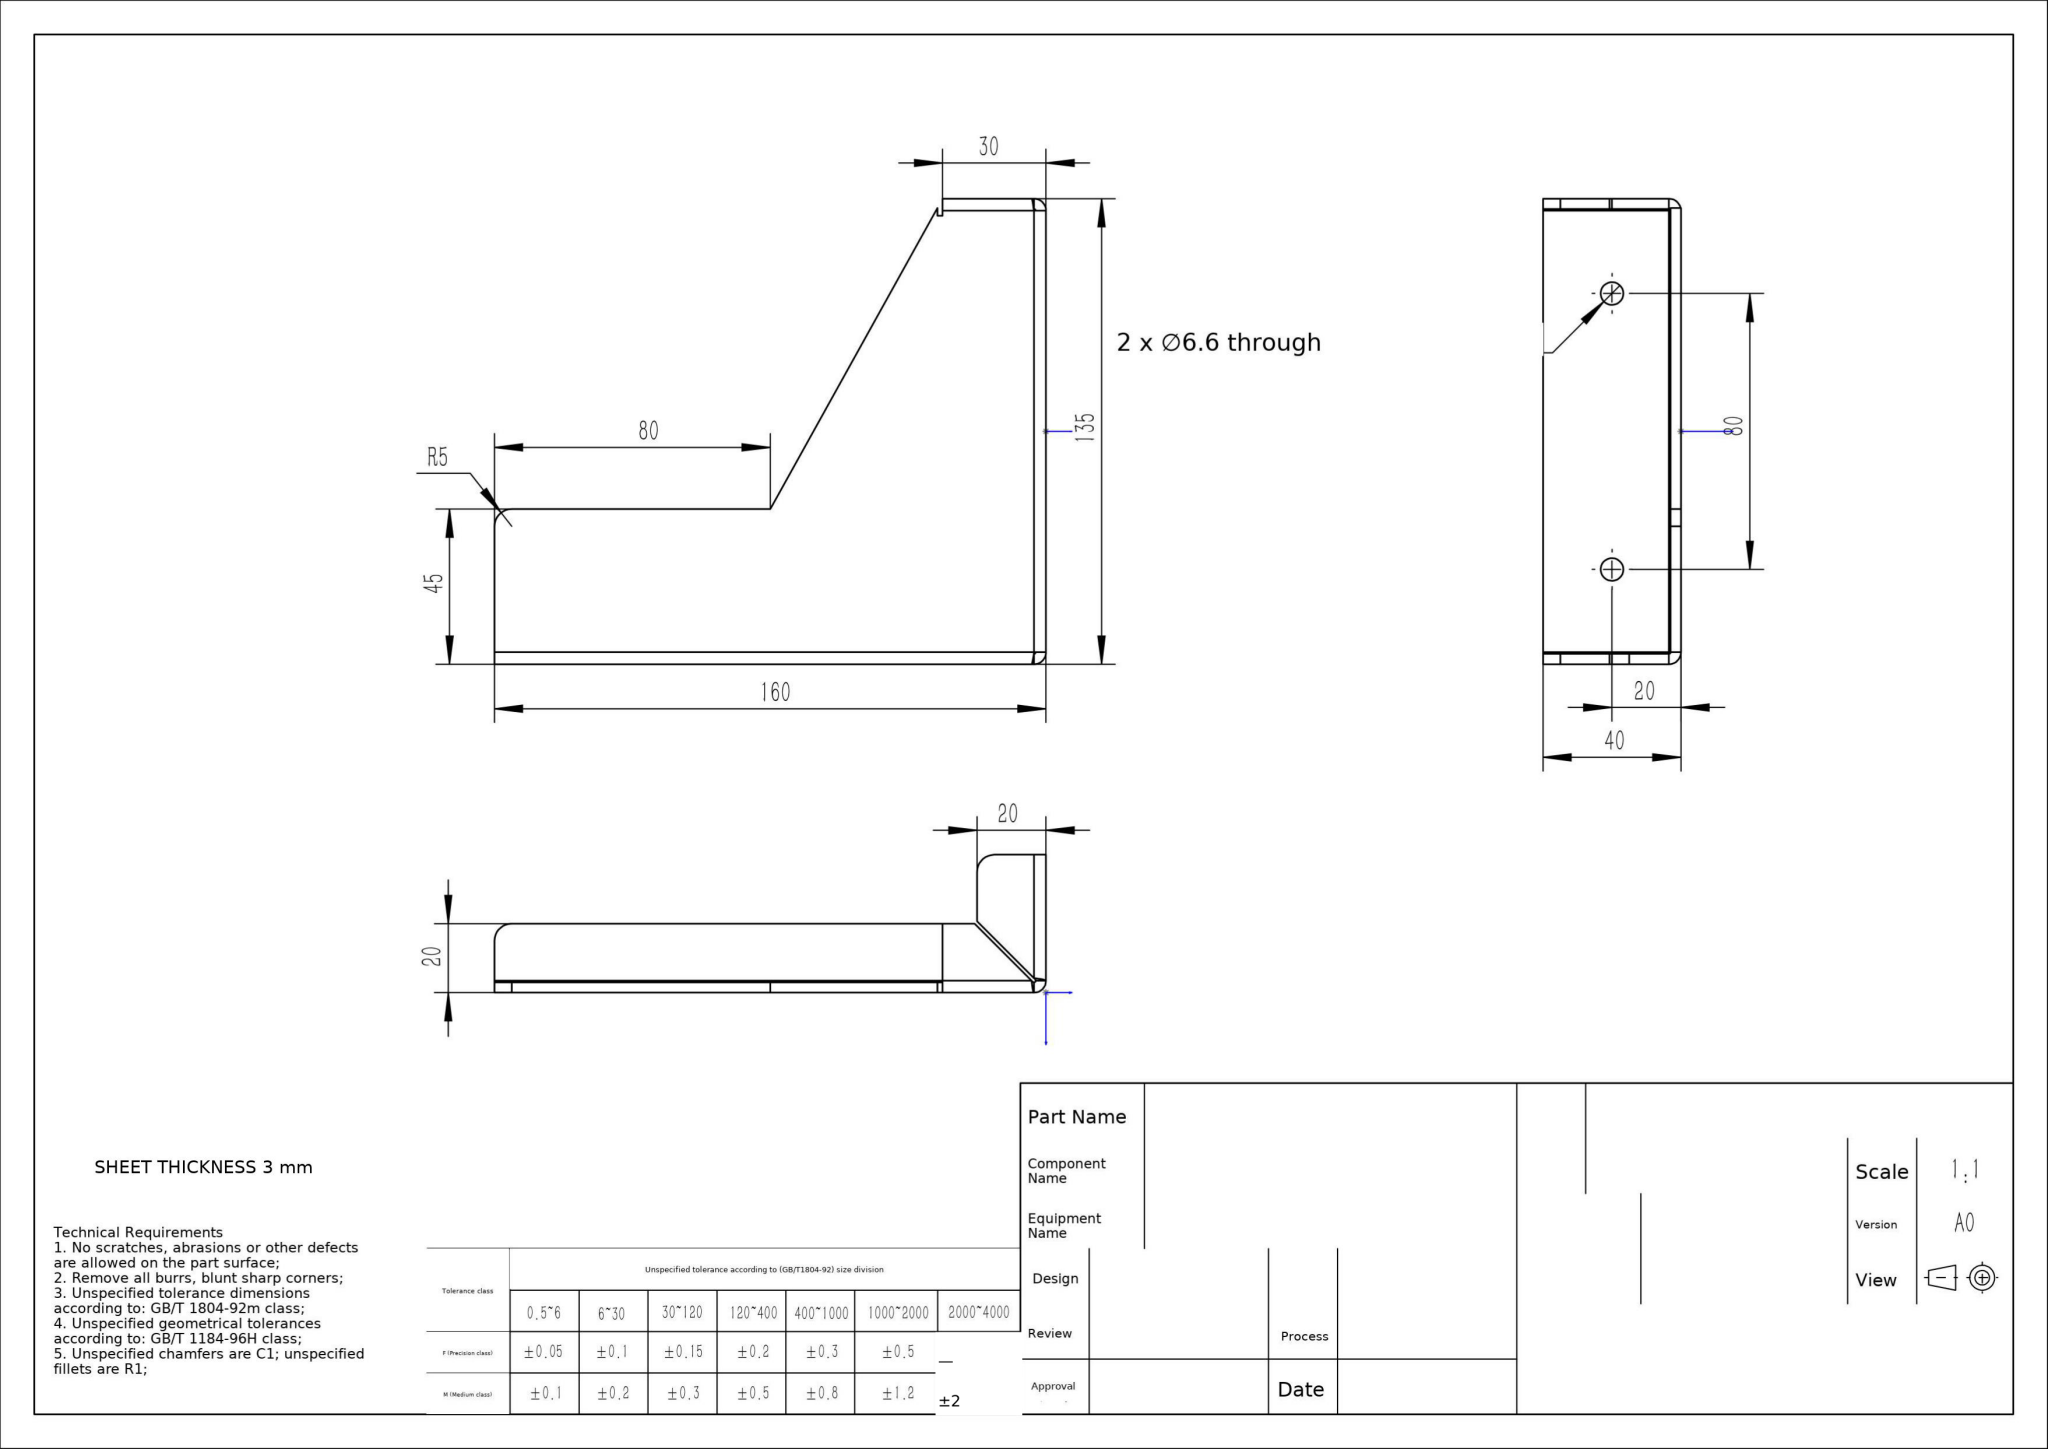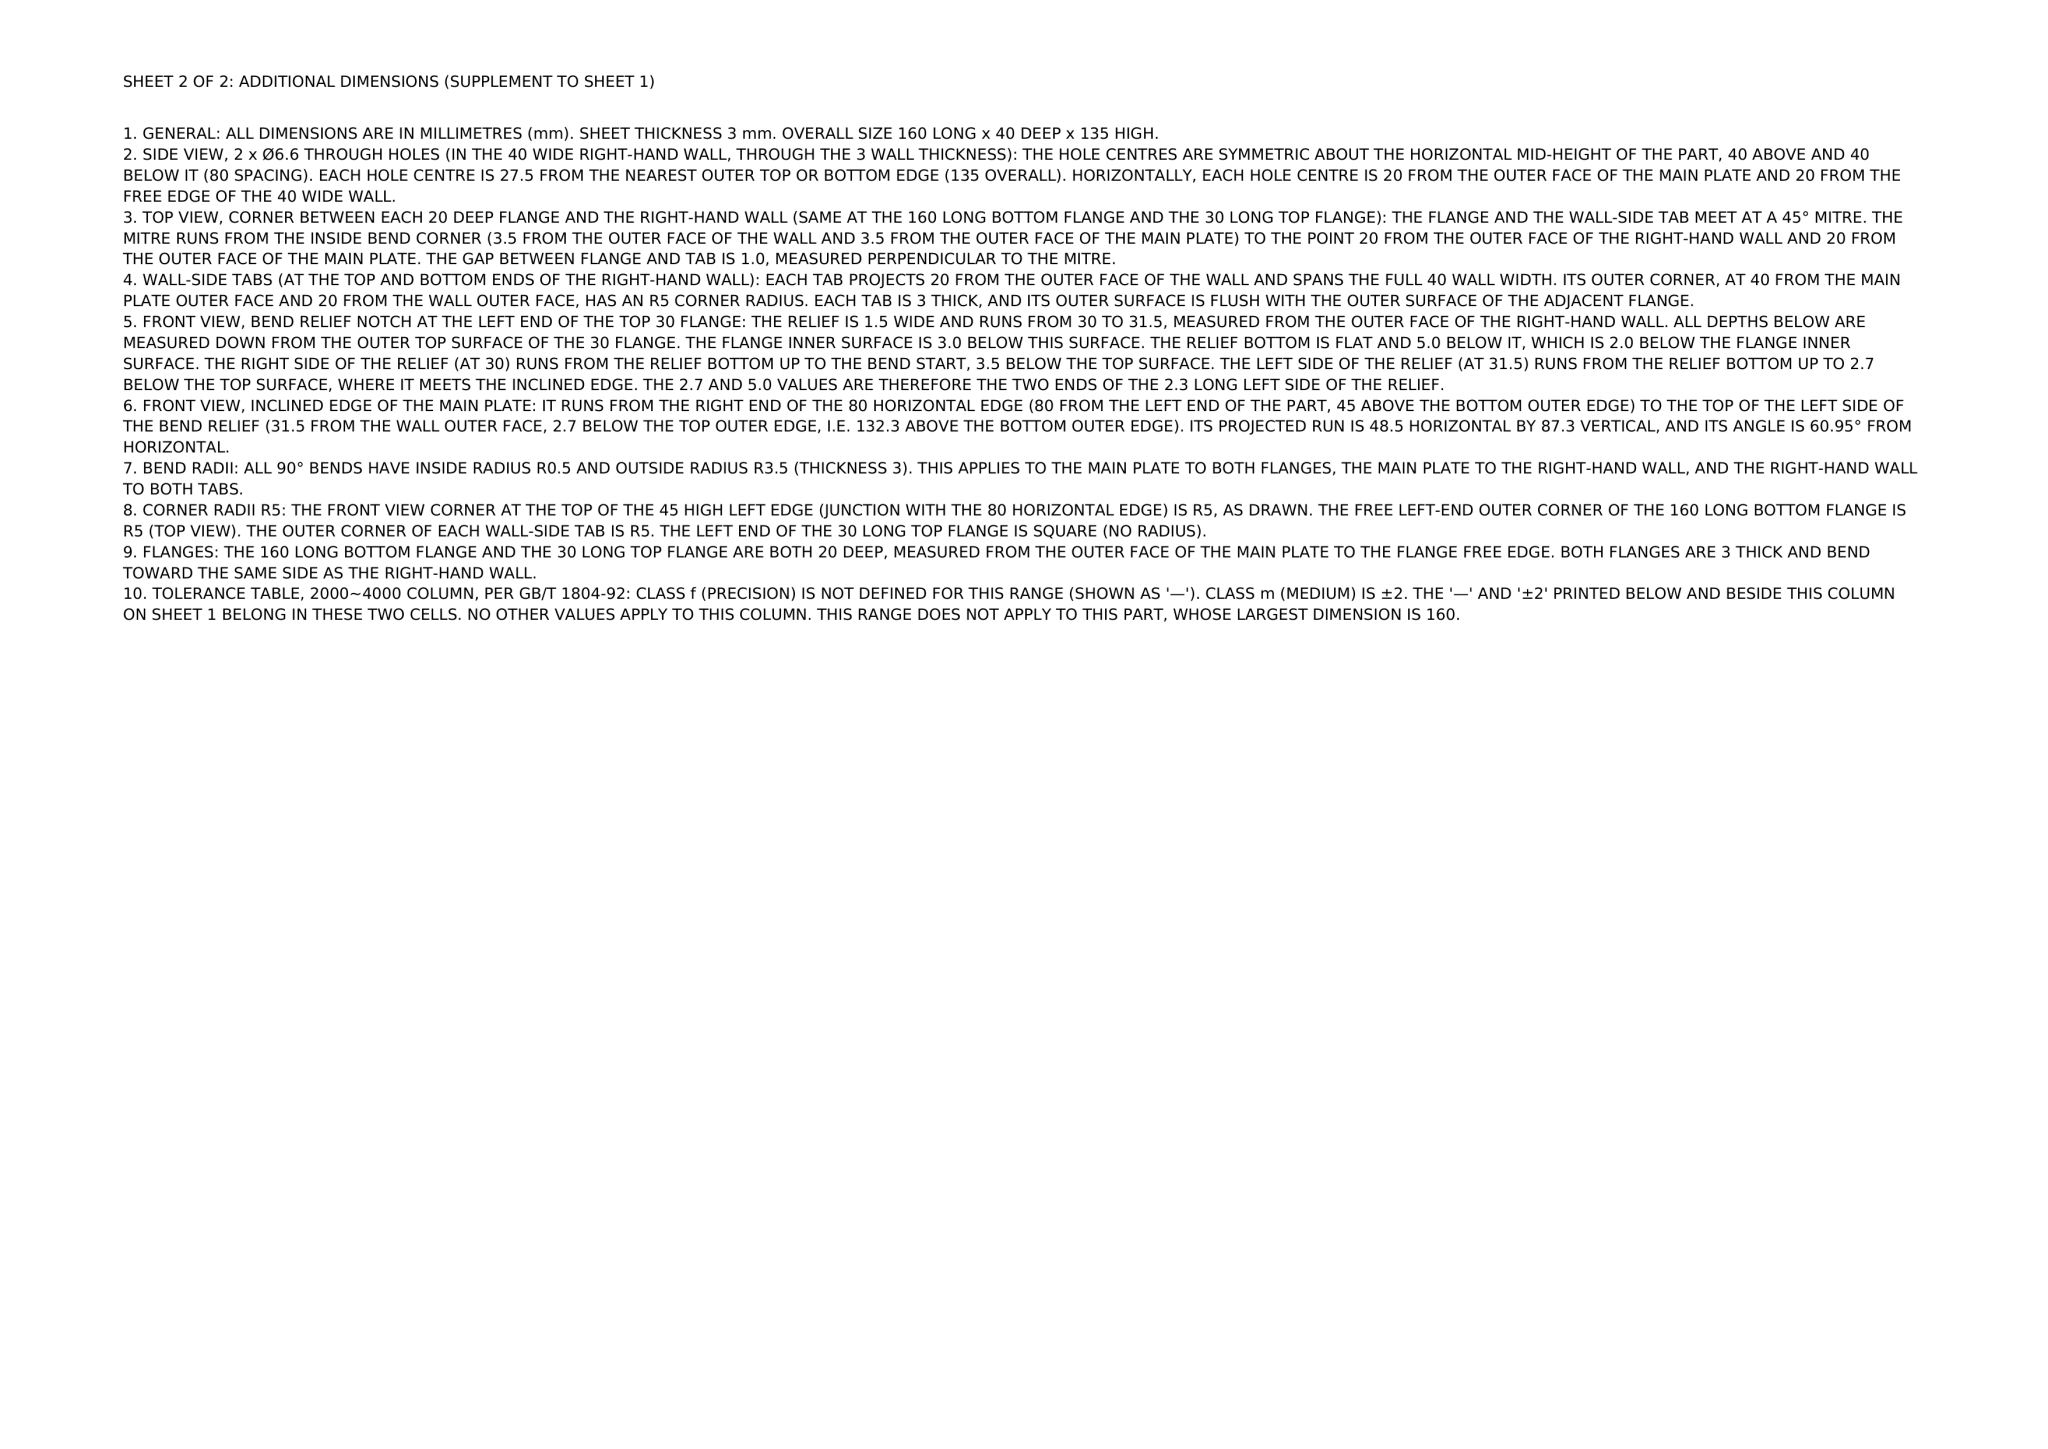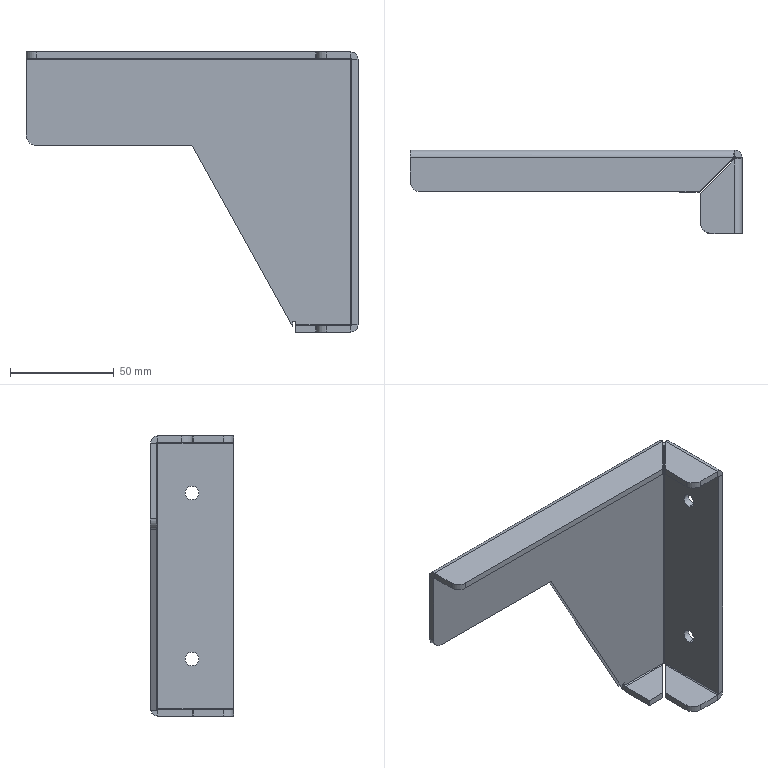Part | NX | mm | Tapered Gusseted Shelf Bracket | 1 solid | 59 faces | box 160 x 40 x 135 mm | volume 61345 mm3 | plane 37 | cylinder 18 | spline 4 | commonest cylinder face diameters 7 x5 1 x5 6.6 x4 10 x4